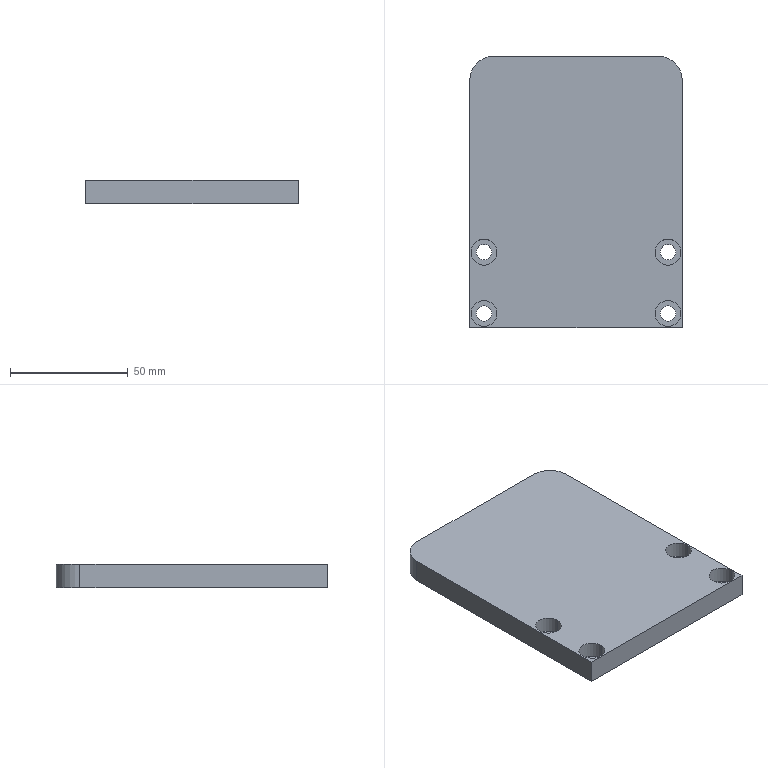Component | SolidWorks | LongSideClampingAssemblyBGeneralAssembly-1_PullFramePlate-0510-1 | 1 solid | 28 faces | box 90 x 115 x 10 mm | volume 100048 mm3 | cylinder 18 | plane 10 | commonest cylinder face diameters 11 x8 6.6 x8 20 x2 | material Q235-A
build123d program:
from build123d import *

# Parameters (mm, degrees)
SKETCH1_W                                          = 90
SKETCH1_H                                          = 115
BOSS_EXTRUDE1_DEPTH                                = 10
HOLE_SIZE_ACCORDING_TO_TYPE_OF_HEX_SOC_D           = 6.6
HOLE_SIZE_ACCORDING_TO_TYPE_OF_HEX_SOC_CBORE_D     = 11
HOLE_SIZE_ACCORDING_TO_TYPE_OF_HEX_SOC_CBORE_DEPTH = 6.8
FILLET1_R                                          = 10


with BuildPart() as part:
    # Sketch1 → Boss-Extrude1 (new body)
    with BuildSketch(Plane.XY):
        Rectangle(SKETCH1_W, SKETCH1_H)
    extrude(amount=BOSS_EXTRUDE1_DEPTH)

    # Hole Size _According to_ Type of Hex Soc (through all)
    with Locations(Plane.XY.offset(10)):
        with Locations((-39, 51.5), (39, 51.5), (-39, 25.5), (39, 25.5)):
            CounterBoreHole(HOLE_SIZE_ACCORDING_TO_TYPE_OF_HEX_SOC_D / 2, HOLE_SIZE_ACCORDING_TO_TYPE_OF_HEX_SOC_CBORE_D / 2, HOLE_SIZE_ACCORDING_TO_TYPE_OF_HEX_SOC_CBORE_DEPTH)

    # Fillet1
    fillet1_edges = [part.edges().sort_by_distance(p)[0] for p in [
        (45, -57.5, 5),
        (-45, -57.5, 5),
    ]]
    fillet(fillet1_edges, radius=FILLET1_R)


solid = part.part

# Placed as in the assembly
solid = solid.moved(Location((-3120.658, -125.109, 3585.5), (0, 0, 180)))
STEP:
#1=COLOUR_RGB('',0.7922,0.8196,0.9333);
#2=FILL_AREA_STYLE_COLOUR('',#1);
#3=FILL_AREA_STYLE('',(#2));
#4=SURFACE_STYLE_FILL_AREA(#3);
#5=SURFACE_SIDE_STYLE('',(#4));
#6=SURFACE_STYLE_USAGE(.BOTH.,#5);
#7=PRESENTATION_STYLE_ASSIGNMENT((#6));
#8=CARTESIAN_POINT('',(-121.109,-6.953,141.287));
#9=VERTEX_POINT('',#8);
#10=CARTESIAN_POINT('',(-121.542,-6.953,141.287));
#11=VERTEX_POINT('',#10);
#12=CARTESIAN_POINT('',(-121.325,-6.953,141.287));
#13=DIRECTION('',(-0.,0.,1.));
#14=DIRECTION('',(-1.,0.,0.));
#15=AXIS2_PLACEMENT_3D('',#12,#13,#14);
#16=CIRCLE('',#15,0.2165);
#17=EDGE_CURVE('',#9,#11,#16,.T.);
#18=ORIENTED_EDGE('',*,*,#17,.F.);
#19=CARTESIAN_POINT('',(-121.109,-6.953,141.555));
#20=VERTEX_POINT('',#19);
#21=CARTESIAN_POINT('',(-121.109,-6.953,141.555));
#22=DIRECTION('',(-0.,0.,1.));
#23=VECTOR('',#22,39.37);
#24=LINE('',#21,#23);
#25=EDGE_CURVE('',#9,#20,#24,.T.);
#26=ORIENTED_EDGE('',*,*,#25,.T.);
#27=CARTESIAN_POINT('',(-121.542,-6.953,141.555));
#28=VERTEX_POINT('',#27);
#29=CARTESIAN_POINT('',(-121.325,-6.953,141.555));
#30=DIRECTION('',(-0.,0.,1.));
#31=DIRECTION('',(-1.,0.,0.));
#32=AXIS2_PLACEMENT_3D('',#29,#30,#31);
#33=CIRCLE('',#32,0.2165);
#34=EDGE_CURVE('',#20,#28,#33,.T.);
#35=ORIENTED_EDGE('',*,*,#34,.T.);
#36=CARTESIAN_POINT('',(-121.542,-6.953,141.555));
#37=DIRECTION('',(-0.,0.,1.));
#38=VECTOR('',#37,39.37);
#39=LINE('',#36,#38);
#40=EDGE_CURVE('',#11,#28,#39,.T.);
#41=ORIENTED_EDGE('',*,*,#40,.F.);
#42=EDGE_LOOP('',(#18,#26,#35,#41));
#43=FACE_OUTER_BOUND('',#42,.T.);
#44=CARTESIAN_POINT('',(-121.325,-6.953,141.555));
#45=DIRECTION('',(-0.,0.,1.));
#46=DIRECTION('',(-1.,0.,0.));
#47=AXIS2_PLACEMENT_3D('',#44,#45,#46);
#48=CYLINDRICAL_SURFACE('',#47,0.2165);
#49=ADVANCED_FACE('',(#43),#48,.F.);
#50=CARTESIAN_POINT('',(-121.195,-6.953,141.161));
#51=VERTEX_POINT('',#50);
#52=CARTESIAN_POINT('',(-121.455,-6.953,141.161));
#53=VERTEX_POINT('',#52);
#54=CARTESIAN_POINT('',(-121.325,-6.953,141.161));
#55=DIRECTION('',(-0.,0.,1.));
#56=DIRECTION('',(-1.,0.,0.));
#57=AXIS2_PLACEMENT_3D('',#54,#55,#56);
#58=CIRCLE('',#57,0.1299);
#59=EDGE_CURVE('',#51,#53,#58,.T.);
#60=ORIENTED_EDGE('',*,*,#59,.F.);
#61=CARTESIAN_POINT('',(-121.195,-6.953,141.287));
#62=VERTEX_POINT('',#61);
#63=CARTESIAN_POINT('',(-121.195,-6.953,141.555));
#64=DIRECTION('',(-0.,0.,1.));
#65=VECTOR('',#64,39.37);
#66=LINE('',#63,#65);
#67=EDGE_CURVE('',#51,#62,#66,.T.);
#68=ORIENTED_EDGE('',*,*,#67,.T.);
#69=CARTESIAN_POINT('',(-121.455,-6.953,141.287));
#70=VERTEX_POINT('',#69);
#71=CARTESIAN_POINT('',(-121.325,-6.953,141.287));
#72=DIRECTION('',(-0.,0.,1.));
#73=DIRECTION('',(-1.,0.,0.));
#74=AXIS2_PLACEMENT_3D('',#71,#72,#73);
#75=CIRCLE('',#74,0.1299);
#76=EDGE_CURVE('',#62,#70,#75,.T.);
#77=ORIENTED_EDGE('',*,*,#76,.T.);
#78=CARTESIAN_POINT('',(-121.455,-6.953,141.555));
#79=DIRECTION('',(-0.,0.,1.));
#80=VECTOR('',#79,39.37);
#81=LINE('',#78,#80);
#82=EDGE_CURVE('',#53,#70,#81,.T.);
#83=ORIENTED_EDGE('',*,*,#82,.F.);
#84=EDGE_LOOP('',(#60,#68,#77,#83));
#85=FACE_OUTER_BOUND('',#84,.T.);
#86=CARTESIAN_POINT('',(-121.325,-6.953,141.555));
#87=DIRECTION('',(-0.,0.,1.));
#88=DIRECTION('',(-1.,0.,0.));
#89=AXIS2_PLACEMENT_3D('',#86,#87,#88);
#90=CYLINDRICAL_SURFACE('',#89,0.1299);
#91=ADVANCED_FACE('',(#85),#90,.F.);
#92=CARTESIAN_POINT('',(-124.179,-6.953,141.287));
#93=VERTEX_POINT('',#92);
#94=CARTESIAN_POINT('',(-124.613,-6.953,141.287));
#95=VERTEX_POINT('',#94);
#96=CARTESIAN_POINT('',(-124.396,-6.953,141.287));
#97=DIRECTION('',(-0.,0.,1.));
#98=DIRECTION('',(-1.,0.,0.));
#99=AXIS2_PLACEMENT_3D('',#96,#97,#98);
#100=CIRCLE('',#99,0.2165);
#101=EDGE_CURVE('',#93,#95,#100,.T.);
#102=ORIENTED_EDGE('',*,*,#101,.F.);
#103=CARTESIAN_POINT('',(-124.179,-6.953,141.555));
#104=VERTEX_POINT('',#103);
#105=CARTESIAN_POINT('',(-124.179,-6.953,141.555));
#106=DIRECTION('',(-0.,0.,1.));
#107=VECTOR('',#106,39.37);
#108=LINE('',#105,#107);
#109=EDGE_CURVE('',#93,#104,#108,.T.);
#110=ORIENTED_EDGE('',*,*,#109,.T.);
#111=CARTESIAN_POINT('',(-124.613,-6.953,141.555));
#112=VERTEX_POINT('',#111);
#113=CARTESIAN_POINT('',(-124.396,-6.953,141.555));
#114=DIRECTION('',(-0.,0.,1.));
#115=DIRECTION('',(-1.,0.,0.));
#116=AXIS2_PLACEMENT_3D('',#113,#114,#115);
#117=CIRCLE('',#116,0.2165);
#118=EDGE_CURVE('',#104,#112,#117,.T.);
#119=ORIENTED_EDGE('',*,*,#118,.T.);
#120=CARTESIAN_POINT('',(-124.613,-6.953,141.555));
#121=DIRECTION('',(-0.,0.,1.));
#122=VECTOR('',#121,39.37);
#123=LINE('',#120,#122);
#124=EDGE_CURVE('',#95,#112,#123,.T.);
#125=ORIENTED_EDGE('',*,*,#124,.F.);
#126=EDGE_LOOP('',(#102,#110,#119,#125));
#127=FACE_OUTER_BOUND('',#126,.T.);
#128=CARTESIAN_POINT('',(-124.396,-6.953,141.555));
#129=DIRECTION('',(-0.,0.,1.));
#130=DIRECTION('',(-1.,0.,0.));
#131=AXIS2_PLACEMENT_3D('',#128,#129,#130);
#132=CYLINDRICAL_SURFACE('',#131,0.2165);
#133=ADVANCED_FACE('',(#127),#132,.F.);
#134=CARTESIAN_POINT('',(-124.266,-6.953,141.161));
#135=VERTEX_POINT('',#134);
#136=CARTESIAN_POINT('',(-124.526,-6.953,141.161));
#137=VERTEX_POINT('',#136);
#138=CARTESIAN_POINT('',(-124.396,-6.953,141.161));
#139=DIRECTION('',(-0.,0.,1.));
#140=DIRECTION('',(-1.,0.,0.));
#141=AXIS2_PLACEMENT_3D('',#138,#139,#140);
#142=CIRCLE('',#141,0.1299);
#143=EDGE_CURVE('',#135,#137,#142,.T.);
#144=ORIENTED_EDGE('',*,*,#143,.F.);
#145=CARTESIAN_POINT('',(-124.266,-6.953,141.287));
#146=VERTEX_POINT('',#145);
#147=CARTESIAN_POINT('',(-124.266,-6.953,141.555));
#148=DIRECTION('',(-0.,0.,1.));
#149=VECTOR('',#148,39.37);
#150=LINE('',#147,#149);
#151=EDGE_CURVE('',#135,#146,#150,.T.);
#152=ORIENTED_EDGE('',*,*,#151,.T.);
#153=CARTESIAN_POINT('',(-124.526,-6.953,141.287));
#154=VERTEX_POINT('',#153);
#155=CARTESIAN_POINT('',(-124.396,-6.953,141.287));
#156=DIRECTION('',(-0.,0.,1.));
#157=DIRECTION('',(-1.,0.,0.));
#158=AXIS2_PLACEMENT_3D('',#155,#156,#157);
#159=CIRCLE('',#158,0.1299);
#160=EDGE_CURVE('',#146,#154,#159,.T.);
#161=ORIENTED_EDGE('',*,*,#160,.T.);
#162=CARTESIAN_POINT('',(-124.526,-6.953,141.555));
#163=DIRECTION('',(-0.,0.,1.));
#164=VECTOR('',#163,39.37);
#165=LINE('',#162,#164);
#166=EDGE_CURVE('',#137,#154,#165,.T.);
#167=ORIENTED_EDGE('',*,*,#166,.F.);
#168=EDGE_LOOP('',(#144,#152,#161,#167));
#169=FACE_OUTER_BOUND('',#168,.T.);
#170=CARTESIAN_POINT('',(-124.396,-6.953,141.555));
#171=DIRECTION('',(-0.,0.,1.));
#172=DIRECTION('',(-1.,0.,0.));
#173=AXIS2_PLACEMENT_3D('',#170,#171,#172);
#174=CYLINDRICAL_SURFACE('',#173,0.1299);
#175=ADVANCED_FACE('',(#169),#174,.F.);
#176=CARTESIAN_POINT('',(-121.109,-5.929,141.287));
#177=VERTEX_POINT('',#176);
#178=CARTESIAN_POINT('',(-121.542,-5.929,141.287));
#179=VERTEX_POINT('',#178);
#180=CARTESIAN_POINT('',(-121.325,-5.929,141.287));
#181=DIRECTION('',(-0.,0.,1.));
#182=DIRECTION('',(-1.,0.,0.));
#183=AXIS2_PLACEMENT_3D('',#180,#181,#182);
#184=CIRCLE('',#183,0.2165);
#185=EDGE_CURVE('',#177,#179,#184,.T.);
#186=ORIENTED_EDGE('',*,*,#185,.F.);
#187=CARTESIAN_POINT('',(-121.109,-5.929,141.555));
#188=VERTEX_POINT('',#187);
#189=CARTESIAN_POINT('',(-121.109,-5.929,141.555));
#190=DIRECTION('',(-0.,0.,1.));
#191=VECTOR('',#190,39.37);
#192=LINE('',#189,#191);
#193=EDGE_CURVE('',#177,#188,#192,.T.);
#194=ORIENTED_EDGE('',*,*,#193,.T.);
#195=CARTESIAN_POINT('',(-121.542,-5.929,141.555));
#196=VERTEX_POINT('',#195);
#197=CARTESIAN_POINT('',(-121.325,-5.929,141.555));
#198=DIRECTION('',(-0.,0.,1.));
#199=DIRECTION('',(-1.,0.,0.));
#200=AXIS2_PLACEMENT_3D('',#197,#198,#199);
#201=CIRCLE('',#200,0.2165);
#202=EDGE_CURVE('',#188,#196,#201,.T.);
#203=ORIENTED_EDGE('',*,*,#202,.T.);
#204=CARTESIAN_POINT('',(-121.542,-5.929,141.555));
#205=DIRECTION('',(-0.,0.,1.));
#206=VECTOR('',#205,39.37);
#207=LINE('',#204,#206);
#208=EDGE_CURVE('',#179,#196,#207,.T.);
#209=ORIENTED_EDGE('',*,*,#208,.F.);
#210=EDGE_LOOP('',(#186,#194,#203,#209));
#211=FACE_OUTER_BOUND('',#210,.T.);
#212=CARTESIAN_POINT('',(-121.325,-5.929,141.555));
#213=DIRECTION('',(-0.,0.,1.));
#214=DIRECTION('',(-1.,0.,0.));
#215=AXIS2_PLACEMENT_3D('',#212,#213,#214);
#216=CYLINDRICAL_SURFACE('',#215,0.2165);
#217=ADVANCED_FACE('',(#211),#216,.F.);
#218=CARTESIAN_POINT('',(-121.195,-5.929,141.161));
#219=VERTEX_POINT('',#218);
#220=CARTESIAN_POINT('',(-121.455,-5.929,141.161));
#221=VERTEX_POINT('',#220);
#222=CARTESIAN_POINT('',(-121.325,-5.929,141.161));
#223=DIRECTION('',(-0.,0.,1.));
#224=DIRECTION('',(-1.,0.,0.));
#225=AXIS2_PLACEMENT_3D('',#222,#223,#224);
#226=CIRCLE('',#225,0.1299);
#227=EDGE_CURVE('',#219,#221,#226,.T.);
#228=ORIENTED_EDGE('',*,*,#227,.F.);
#229=CARTESIAN_POINT('',(-121.195,-5.929,141.287));
#230=VERTEX_POINT('',#229);
#231=CARTESIAN_POINT('',(-121.195,-5.929,141.555));
#232=DIRECTION('',(-0.,0.,1.));
#233=VECTOR('',#232,39.37);
#234=LINE('',#231,#233);
#235=EDGE_CURVE('',#219,#230,#234,.T.);
#236=ORIENTED_EDGE('',*,*,#235,.T.);
#237=CARTESIAN_POINT('',(-121.455,-5.929,141.287));
#238=VERTEX_POINT('',#237);
#239=CARTESIAN_POINT('',(-121.325,-5.929,141.287));
#240=DIRECTION('',(-0.,0.,1.));
#241=DIRECTION('',(-1.,0.,0.));
#242=AXIS2_PLACEMENT_3D('',#239,#240,#241);
#243=CIRCLE('',#242,0.1299);
#244=EDGE_CURVE('',#230,#238,#243,.T.);
#245=ORIENTED_EDGE('',*,*,#244,.T.);
#246=CARTESIAN_POINT('',(-121.455,-5.929,141.555));
#247=DIRECTION('',(-0.,0.,1.));
#248=VECTOR('',#247,39.37);
#249=LINE('',#246,#248);
#250=EDGE_CURVE('',#221,#238,#249,.T.);
#251=ORIENTED_EDGE('',*,*,#250,.F.);
#252=EDGE_LOOP('',(#228,#236,#245,#251));
#253=FACE_OUTER_BOUND('',#252,.T.);
#254=CARTESIAN_POINT('',(-121.325,-5.929,141.555));
#255=DIRECTION('',(-0.,0.,1.));
#256=DIRECTION('',(-1.,0.,0.));
#257=AXIS2_PLACEMENT_3D('',#254,#255,#256);
#258=CYLINDRICAL_SURFACE('',#257,0.1299);
#259=ADVANCED_FACE('',(#253),#258,.F.);
#260=CARTESIAN_POINT('',(-124.179,-5.929,141.287));
#261=VERTEX_POINT('',#260);
#262=CARTESIAN_POINT('',(-124.613,-5.929,141.287));
#263=VERTEX_POINT('',#262);
#264=CARTESIAN_POINT('',(-124.396,-5.929,141.287));
#265=DIRECTION('',(-0.,0.,1.));
#266=DIRECTION('',(-1.,0.,0.));
#267=AXIS2_PLACEMENT_3D('',#264,#265,#266);
#268=CIRCLE('',#267,0.2165);
#269=EDGE_CURVE('',#261,#263,#268,.T.);
#270=ORIENTED_EDGE('',*,*,#269,.F.);
#271=CARTESIAN_POINT('',(-124.179,-5.929,141.555));
#272=VERTEX_POINT('',#271);
#273=CARTESIAN_POINT('',(-124.179,-5.929,141.555));
#274=DIRECTION('',(-0.,0.,1.));
#275=VECTOR('',#274,39.37);
#276=LINE('',#273,#275);
#277=EDGE_CURVE('',#261,#272,#276,.T.);
#278=ORIENTED_EDGE('',*,*,#277,.T.);
#279=CARTESIAN_POINT('',(-124.613,-5.929,141.555));
#280=VERTEX_POINT('',#279);
#281=CARTESIAN_POINT('',(-124.396,-5.929,141.555));
#282=DIRECTION('',(-0.,0.,1.));
#283=DIRECTION('',(-1.,0.,0.));
#284=AXIS2_PLACEMENT_3D('',#281,#282,#283);
#285=CIRCLE('',#284,0.2165);
#286=EDGE_CURVE('',#272,#280,#285,.T.);
#287=ORIENTED_EDGE('',*,*,#286,.T.);
#288=CARTESIAN_POINT('',(-124.613,-5.929,141.555));
#289=DIRECTION('',(-0.,0.,1.));
#290=VECTOR('',#289,39.37);
#291=LINE('',#288,#290);
#292=EDGE_CURVE('',#263,#280,#291,.T.);
#293=ORIENTED_EDGE('',*,*,#292,.F.);
#294=EDGE_LOOP('',(#270,#278,#287,#293));
#295=FACE_OUTER_BOUND('',#294,.T.);
#296=CARTESIAN_POINT('',(-124.396,-5.929,141.555));
#297=DIRECTION('',(-0.,0.,1.));
#298=DIRECTION('',(-1.,0.,0.));
#299=AXIS2_PLACEMENT_3D('',#296,#297,#298);
#300=CYLINDRICAL_SURFACE('',#299,0.2165);
#301=ADVANCED_FACE('',(#295),#300,.F.);
#302=CARTESIAN_POINT('',(-124.266,-5.929,141.161));
#303=VERTEX_POINT('',#302);
#304=CARTESIAN_POINT('',(-124.526,-5.929,141.161));
#305=VERTEX_POINT('',#304);
#306=CARTESIAN_POINT('',(-124.396,-5.929,141.161));
#307=DIRECTION('',(-0.,0.,1.));
#308=DIRECTION('',(-1.,0.,0.));
#309=AXIS2_PLACEMENT_3D('',#306,#307,#308);
#310=CIRCLE('',#309,0.1299);
#311=EDGE_CURVE('',#303,#305,#310,.T.);
#312=ORIENTED_EDGE('',*,*,#311,.F.);
#313=CARTESIAN_POINT('',(-124.266,-5.929,141.287));
#314=VERTEX_POINT('',#313);
#315=CARTESIAN_POINT('',(-124.266,-5.929,141.555));
#316=DIRECTION('',(-0.,0.,1.));
#317=VECTOR('',#316,39.37);
#318=LINE('',#315,#317);
#319=EDGE_CURVE('',#303,#314,#318,.T.);
#320=ORIENTED_EDGE('',*,*,#319,.T.);
#321=CARTESIAN_POINT('',(-124.526,-5.929,141.287));
#322=VERTEX_POINT('',#321);
#323=CARTESIAN_POINT('',(-124.396,-5.929,141.287));
#324=DIRECTION('',(-0.,0.,1.));
#325=DIRECTION('',(-1.,0.,0.));
#326=AXIS2_PLACEMENT_3D('',#323,#324,#325);
#327=CIRCLE('',#326,0.1299);
#328=EDGE_CURVE('',#314,#322,#327,.T.);
#329=ORIENTED_EDGE('',*,*,#328,.T.);
#330=CARTESIAN_POINT('',(-124.526,-5.929,141.555));
#331=DIRECTION('',(-0.,0.,1.));
#332=VECTOR('',#331,39.37);
#333=LINE('',#330,#332);
#334=EDGE_CURVE('',#305,#322,#333,.T.);
#335=ORIENTED_EDGE('',*,*,#334,.F.);
#336=EDGE_LOOP('',(#312,#320,#329,#335));
#337=FACE_OUTER_BOUND('',#336,.T.);
#338=CARTESIAN_POINT('',(-124.396,-5.929,141.555));
#339=DIRECTION('',(-0.,0.,1.));
#340=DIRECTION('',(-1.,0.,0.));
#341=AXIS2_PLACEMENT_3D('',#338,#339,#340);
#342=CYLINDRICAL_SURFACE('',#341,0.1299);
#343=ADVANCED_FACE('',(#337),#342,.F.);
#344=CARTESIAN_POINT('',(-124.632,-3.055,141.555));
#345=VERTEX_POINT('',#344);
#346=CARTESIAN_POINT('',(-124.632,-7.189,141.555));
#347=VERTEX_POINT('',#346);
#348=CARTESIAN_POINT('',(-124.632,-2.662,141.555));
#349=DIRECTION('',(-0.,-1.,0.));
#350=VECTOR('',#349,39.37);
#351=LINE('',#348,#350);
#352=EDGE_CURVE('',#345,#347,#351,.T.);
#353=ORIENTED_EDGE('',*,*,#352,.F.);
#354=CARTESIAN_POINT('',(-124.632,-3.055,141.161));
#355=VERTEX_POINT('',#354);
#356=CARTESIAN_POINT('',(-124.632,-3.055,141.555));
#357=DIRECTION('',(0.,-0.,-1.));
#358=VECTOR('',#357,39.37);
#359=LINE('',#356,#358);
#360=EDGE_CURVE('',#345,#355,#359,.T.);
#361=ORIENTED_EDGE('',*,*,#360,.T.);
#362=CARTESIAN_POINT('',(-124.632,-7.189,141.161));
#363=VERTEX_POINT('',#362);
#364=CARTESIAN_POINT('',(-124.632,-2.662,141.161));
#365=DIRECTION('',(-0.,-1.,0.));
#366=VECTOR('',#365,39.37);
#367=LINE('',#364,#366);
#368=EDGE_CURVE('',#355,#363,#367,.T.);
#369=ORIENTED_EDGE('',*,*,#368,.T.);
#370=CARTESIAN_POINT('',(-124.632,-7.189,141.555));
#371=DIRECTION('',(0.,-0.,-1.));
#372=VECTOR('',#371,39.37);
#373=LINE('',#370,#372);
#374=EDGE_CURVE('',#347,#363,#373,.T.);
#375=ORIENTED_EDGE('',*,*,#374,.F.);
#376=EDGE_LOOP('',(#353,#361,#369,#375));
#377=FACE_OUTER_BOUND('',#376,.T.);
#378=CARTESIAN_POINT('',(-124.632,-2.662,141.555));
#379=DIRECTION('',(1.,-0.,0.));
#380=DIRECTION('',(-0.,0.,1.));
#381=AXIS2_PLACEMENT_3D('',#378,#379,#380);
#382=PLANE('',#381);
#383=ADVANCED_FACE('',(#377),#382,.F.);
#384=CARTESIAN_POINT('',(-121.089,-7.189,141.161));
#385=VERTEX_POINT('',#384);
#386=CARTESIAN_POINT('',(-121.089,-7.189,141.161));
#387=DIRECTION('',(1.,-0.,0.));
#388=VECTOR('',#387,39.37);
#389=LINE('',#386,#388);
#390=EDGE_CURVE('',#363,#385,#389,.T.);
#391=ORIENTED_EDGE('',*,*,#390,.T.);
#392=CARTESIAN_POINT('',(-121.089,-7.189,141.555));
#393=VERTEX_POINT('',#392);
#394=CARTESIAN_POINT('',(-121.089,-7.189,141.555));
#395=DIRECTION('',(0.,-0.,-1.));
#396=VECTOR('',#395,39.37);
#397=LINE('',#394,#396);
#398=EDGE_CURVE('',#393,#385,#397,.T.);
#399=ORIENTED_EDGE('',*,*,#398,.F.);
#400=CARTESIAN_POINT('',(-121.089,-7.189,141.555));
#401=DIRECTION('',(1.,-0.,0.));
#402=VECTOR('',#401,39.37);
#403=LINE('',#400,#402);
#404=EDGE_CURVE('',#347,#393,#403,.T.);
#405=ORIENTED_EDGE('',*,*,#404,.F.);
#406=ORIENTED_EDGE('',*,*,#374,.T.);
#407=EDGE_LOOP('',(#391,#399,#405,#406));
#408=FACE_OUTER_BOUND('',#407,.T.);
#409=CARTESIAN_POINT('',(-121.089,-7.189,141.555));
#410=DIRECTION('',(0.,1.,-0.));
#411=DIRECTION('',(0.,-0.,-1.));
#412=AXIS2_PLACEMENT_3D('',#409,#410,#411);
#413=PLANE('',#412);
#414=ADVANCED_FACE('',(#408),#413,.F.);
#415=CARTESIAN_POINT('',(-121.089,-3.055,141.161));
#416=VERTEX_POINT('',#415);
#417=CARTESIAN_POINT('',(-121.089,-2.662,141.161));
#418=DIRECTION('',(0.,1.,-0.));
#419=VECTOR('',#418,39.37);
#420=LINE('',#417,#419);
#421=EDGE_CURVE('',#385,#416,#420,.T.);
#422=ORIENTED_EDGE('',*,*,#421,.T.);
#423=CARTESIAN_POINT('',(-121.089,-3.055,141.555));
#424=VERTEX_POINT('',#423);
#425=CARTESIAN_POINT('',(-121.089,-3.055,141.555));
#426=DIRECTION('',(-0.,0.,1.));
#427=VECTOR('',#426,39.37);
#428=LINE('',#425,#427);
#429=EDGE_CURVE('',#416,#424,#428,.T.);
#430=ORIENTED_EDGE('',*,*,#429,.T.);
#431=CARTESIAN_POINT('',(-121.089,-2.662,141.555));
#432=DIRECTION('',(0.,1.,-0.));
#433=VECTOR('',#432,39.37);
#434=LINE('',#431,#433);
#435=EDGE_CURVE('',#393,#424,#434,.T.);
#436=ORIENTED_EDGE('',*,*,#435,.F.);
#437=ORIENTED_EDGE('',*,*,#398,.T.);
#438=EDGE_LOOP('',(#422,#430,#436,#437));
#439=FACE_OUTER_BOUND('',#438,.T.);
#440=CARTESIAN_POINT('',(-121.089,-2.662,141.555));
#441=DIRECTION('',(-1.,0.,-0.));
#442=DIRECTION('',(0.,-0.,-1.));
#443=AXIS2_PLACEMENT_3D('',#440,#441,#442);
#444=PLANE('',#443);
#445=ADVANCED_FACE('',(#439),#444,.F.);
#446=CARTESIAN_POINT('',(-121.483,-2.662,141.555));
#447=VERTEX_POINT('',#446);
#448=CARTESIAN_POINT('',(-124.239,-2.662,141.555));
#449=VERTEX_POINT('',#448);
#450=CARTESIAN_POINT('',(-121.089,-2.662,141.555));
#451=DIRECTION('',(-1.,0.,-0.));
#452=VECTOR('',#451,39.37);
#453=LINE('',#450,#452);
#454=EDGE_CURVE('',#447,#449,#453,.T.);
#455=ORIENTED_EDGE('',*,*,#454,.F.);
#456=CARTESIAN_POINT('',(-121.483,-2.662,141.161));
#457=VERTEX_POINT('',#456);
#458=CARTESIAN_POINT('',(-121.483,-2.662,141.555));
#459=DIRECTION('',(0.,-0.,-1.));
#460=VECTOR('',#459,39.37);
#461=LINE('',#458,#460);
#462=EDGE_CURVE('',#447,#457,#461,.T.);
#463=ORIENTED_EDGE('',*,*,#462,.T.);
#464=CARTESIAN_POINT('',(-124.239,-2.662,141.161));
#465=VERTEX_POINT('',#464);
#466=CARTESIAN_POINT('',(-121.089,-2.662,141.161));
#467=DIRECTION('',(-1.,0.,-0.));
#468=VECTOR('',#467,39.37);
#469=LINE('',#466,#468);
#470=EDGE_CURVE('',#457,#465,#469,.T.);
#471=ORIENTED_EDGE('',*,*,#470,.T.);
#472=CARTESIAN_POINT('',(-124.239,-2.662,141.555));
#473=DIRECTION('',(-0.,0.,1.));
#474=VECTOR('',#473,39.37);
#475=LINE('',#472,#474);
#476=EDGE_CURVE('',#465,#449,#475,.T.);
#477=ORIENTED_EDGE('',*,*,#476,.T.);
#478=EDGE_LOOP('',(#455,#463,#471,#477));
#479=FACE_OUTER_BOUND('',#478,.T.);
#480=CARTESIAN_POINT('',(-121.089,-2.662,141.555));
#481=DIRECTION('',(-0.,-1.,0.));
#482=DIRECTION('',(-0.,0.,1.));
#483=AXIS2_PLACEMENT_3D('',#480,#481,#482);
#484=PLANE('',#483);
#485=ADVANCED_FACE('',(#479),#484,.F.);
#486=CARTESIAN_POINT('',(-121.325,-6.953,141.555));
#487=DIRECTION('',(-0.,0.,1.));
#488=DIRECTION('',(-1.,0.,0.));
#489=AXIS2_PLACEMENT_3D('',#486,#487,#488);
#490=CIRCLE('',#489,0.2165);
#491=EDGE_CURVE('',#28,#20,#490,.T.);
#492=ORIENTED_EDGE('',*,*,#491,.F.);
#493=ORIENTED_EDGE('',*,*,#34,.F.);
#494=EDGE_LOOP('',(#492,#493));
#495=FACE_BOUND('',#494,.T.);
#496=CARTESIAN_POINT('',(-124.396,-6.953,141.555));
#497=DIRECTION('',(-0.,0.,1.));
#498=DIRECTION('',(-1.,0.,0.));
#499=AXIS2_PLACEMENT_3D('',#496,#497,#498);
#500=CIRCLE('',#499,0.2165);
#501=EDGE_CURVE('',#112,#104,#500,.T.);
#502=ORIENTED_EDGE('',*,*,#501,.F.);
#503=ORIENTED_EDGE('',*,*,#118,.F.);
#504=EDGE_LOOP('',(#502,#503));
#505=FACE_BOUND('',#504,.T.);
#506=CARTESIAN_POINT('',(-121.325,-5.929,141.555));
#507=DIRECTION('',(-0.,0.,1.));
#508=DIRECTION('',(-1.,0.,0.));
#509=AXIS2_PLACEMENT_3D('',#506,#507,#508);
#510=CIRCLE('',#509,0.2165);
#511=EDGE_CURVE('',#196,#188,#510,.T.);
#512=ORIENTED_EDGE('',*,*,#511,.F.);
#513=ORIENTED_EDGE('',*,*,#202,.F.);
#514=EDGE_LOOP('',(#512,#513));
#515=FACE_BOUND('',#514,.T.);
#516=CARTESIAN_POINT('',(-124.396,-5.929,141.555));
#517=DIRECTION('',(-0.,0.,1.));
#518=DIRECTION('',(-1.,0.,0.));
#519=AXIS2_PLACEMENT_3D('',#516,#517,#518);
#520=CIRCLE('',#519,0.2165);
#521=EDGE_CURVE('',#280,#272,#520,.T.);
#522=ORIENTED_EDGE('',*,*,#521,.F.);
#523=ORIENTED_EDGE('',*,*,#286,.F.);
#524=EDGE_LOOP('',(#522,#523));
#525=FACE_BOUND('',#524,.T.);
#526=ORIENTED_EDGE('',*,*,#435,.T.);
#527=CARTESIAN_POINT('',(-121.483,-3.055,141.555));
#528=DIRECTION('',(-0.,0.,1.));
#529=DIRECTION('',(1.,-0.,0.));
#530=AXIS2_PLACEMENT_3D('',#527,#528,#529);
#531=CIRCLE('',#530,0.3937);
#532=EDGE_CURVE('',#424,#447,#531,.T.);
#533=ORIENTED_EDGE('',*,*,#532,.T.);
#534=ORIENTED_EDGE('',*,*,#454,.T.);
#535=CARTESIAN_POINT('',(-124.239,-3.055,141.555));
#536=DIRECTION('',(-0.,0.,1.));
#537=DIRECTION('',(1.,-0.,0.));
#538=AXIS2_PLACEMENT_3D('',#535,#536,#537);
#539=CIRCLE('',#538,0.3937);
#540=EDGE_CURVE('',#449,#345,#539,.T.);
#541=ORIENTED_EDGE('',*,*,#540,.T.);
#542=ORIENTED_EDGE('',*,*,#352,.T.);
#543=ORIENTED_EDGE('',*,*,#404,.T.);
#544=EDGE_LOOP('',(#526,#533,#534,#541,#542,#543));
#545=FACE_OUTER_BOUND('',#544,.T.);
#546=CARTESIAN_POINT('',(-122.861,-4.926,141.555));
#547=DIRECTION('',(0.,-0.,-1.));
#548=DIRECTION('',(1.,-0.,0.));
#549=AXIS2_PLACEMENT_3D('',#546,#547,#548);
#550=PLANE('',#549);
#551=ADVANCED_FACE('',(#495,#505,#515,#525,#545),#550,.F.);
#552=CARTESIAN_POINT('',(-121.325,-6.953,141.161));
#553=DIRECTION('',(-0.,0.,1.));
#554=DIRECTION('',(-1.,0.,0.));
#555=AXIS2_PLACEMENT_3D('',#552,#553,#554);
#556=CIRCLE('',#555,0.1299);
#557=EDGE_CURVE('',#53,#51,#556,.T.);
#558=ORIENTED_EDGE('',*,*,#557,.T.);
#559=ORIENTED_EDGE('',*,*,#59,.T.);
#560=EDGE_LOOP('',(#558,#559));
#561=FACE_BOUND('',#560,.T.);
#562=CARTESIAN_POINT('',(-124.396,-6.953,141.161));
#563=DIRECTION('',(-0.,0.,1.));
#564=DIRECTION('',(-1.,0.,0.));
#565=AXIS2_PLACEMENT_3D('',#562,#563,#564);
#566=CIRCLE('',#565,0.1299);
#567=EDGE_CURVE('',#137,#135,#566,.T.);
#568=ORIENTED_EDGE('',*,*,#567,.T.);
#569=ORIENTED_EDGE('',*,*,#143,.T.);
#570=EDGE_LOOP('',(#568,#569));
#571=FACE_BOUND('',#570,.T.);
#572=CARTESIAN_POINT('',(-121.325,-5.929,141.161));
#573=DIRECTION('',(-0.,0.,1.));
#574=DIRECTION('',(-1.,0.,0.));
#575=AXIS2_PLACEMENT_3D('',#572,#573,#574);
#576=CIRCLE('',#575,0.1299);
#577=EDGE_CURVE('',#221,#219,#576,.T.);
#578=ORIENTED_EDGE('',*,*,#577,.T.);
#579=ORIENTED_EDGE('',*,*,#227,.T.);
#580=EDGE_LOOP('',(#578,#579));
#581=FACE_BOUND('',#580,.T.);
#582=CARTESIAN_POINT('',(-124.396,-5.929,141.161));
#583=DIRECTION('',(-0.,0.,1.));
#584=DIRECTION('',(-1.,0.,0.));
#585=AXIS2_PLACEMENT_3D('',#582,#583,#584);
#586=CIRCLE('',#585,0.1299);
#587=EDGE_CURVE('',#305,#303,#586,.T.);
#588=ORIENTED_EDGE('',*,*,#587,.T.);
#589=ORIENTED_EDGE('',*,*,#311,.T.);
#590=EDGE_LOOP('',(#588,#589));
#591=FACE_BOUND('',#590,.T.);
#592=ORIENTED_EDGE('',*,*,#470,.F.);
#593=CARTESIAN_POINT('',(-121.483,-3.055,141.161));
#594=DIRECTION('',(0.,-0.,-1.));
#595=DIRECTION('',(1.,-0.,0.));
#596=AXIS2_PLACEMENT_3D('',#593,#594,#595);
#597=CIRCLE('',#596,0.3937);
#598=EDGE_CURVE('',#457,#416,#597,.T.);
#599=ORIENTED_EDGE('',*,*,#598,.T.);
#600=ORIENTED_EDGE('',*,*,#421,.F.);
#601=ORIENTED_EDGE('',*,*,#390,.F.);
#602=ORIENTED_EDGE('',*,*,#368,.F.);
#603=CARTESIAN_POINT('',(-124.239,-3.055,141.161));
#604=DIRECTION('',(0.,-0.,-1.));
#605=DIRECTION('',(1.,-0.,0.));
#606=AXIS2_PLACEMENT_3D('',#603,#604,#605);
#607=CIRCLE('',#606,0.3937);
#608=EDGE_CURVE('',#355,#465,#607,.T.);
#609=ORIENTED_EDGE('',*,*,#608,.T.);
#610=EDGE_LOOP('',(#592,#599,#600,#601,#602,#609));
#611=FACE_OUTER_BOUND('',#610,.T.);
#612=CARTESIAN_POINT('',(-122.861,-4.926,141.161));
#613=DIRECTION('',(0.,-0.,-1.));
#614=DIRECTION('',(1.,-0.,0.));
#615=AXIS2_PLACEMENT_3D('',#612,#613,#614);
#616=PLANE('',#615);
#617=ADVANCED_FACE('',(#561,#571,#581,#591,#611),#616,.T.);
#618=ORIENTED_EDGE('',*,*,#319,.F.);
#619=ORIENTED_EDGE('',*,*,#587,.F.);
#620=ORIENTED_EDGE('',*,*,#334,.T.);
#621=CARTESIAN_POINT('',(-124.396,-5.929,141.287));
#622=DIRECTION('',(-0.,0.,1.));
#623=DIRECTION('',(-1.,0.,0.));
#624=AXIS2_PLACEMENT_3D('',#621,#622,#623);
#625=CIRCLE('',#624,0.1299);
#626=EDGE_CURVE('',#322,#314,#625,.T.);
#627=ORIENTED_EDGE('',*,*,#626,.T.);
#628=EDGE_LOOP('',(#618,#619,#620,#627));
#629=FACE_OUTER_BOUND('',#628,.T.);
#630=CARTESIAN_POINT('',(-124.396,-5.929,141.555));
#631=DIRECTION('',(-0.,0.,1.));
#632=DIRECTION('',(-1.,0.,0.));
#633=AXIS2_PLACEMENT_3D('',#630,#631,#632);
#634=CYLINDRICAL_SURFACE('',#633,0.1299);
#635=ADVANCED_FACE('',(#629),#634,.F.);
#636=ORIENTED_EDGE('',*,*,#626,.F.);
#637=ORIENTED_EDGE('',*,*,#328,.F.);
#638=EDGE_LOOP('',(#636,#637));
#639=FACE_BOUND('',#638,.T.);
#640=CARTESIAN_POINT('',(-124.396,-5.929,141.287));
#641=DIRECTION('',(-0.,0.,1.));
#642=DIRECTION('',(-1.,0.,0.));
#643=AXIS2_PLACEMENT_3D('',#640,#641,#642);
#644=CIRCLE('',#643,0.2165);
#645=EDGE_CURVE('',#263,#261,#644,.T.);
#646=ORIENTED_EDGE('',*,*,#645,.T.);
#647=ORIENTED_EDGE('',*,*,#269,.T.);
#648=EDGE_LOOP('',(#646,#647));
#649=FACE_OUTER_BOUND('',#648,.T.);
#650=CARTESIAN_POINT('',(-124.526,-5.929,141.287));
#651=DIRECTION('',(0.,-0.,-1.));
#652=DIRECTION('',(1.,-0.,0.));
#653=AXIS2_PLACEMENT_3D('',#650,#651,#652);
#654=PLANE('',#653);
#655=ADVANCED_FACE('',(#639,#649),#654,.F.);
#656=ORIENTED_EDGE('',*,*,#277,.F.);
#657=ORIENTED_EDGE('',*,*,#645,.F.);
#658=ORIENTED_EDGE('',*,*,#292,.T.);
#659=ORIENTED_EDGE('',*,*,#521,.T.);
#660=EDGE_LOOP('',(#656,#657,#658,#659));
#661=FACE_OUTER_BOUND('',#660,.T.);
#662=CARTESIAN_POINT('',(-124.396,-5.929,141.555));
#663=DIRECTION('',(-0.,0.,1.));
#664=DIRECTION('',(-1.,0.,0.));
#665=AXIS2_PLACEMENT_3D('',#662,#663,#664);
#666=CYLINDRICAL_SURFACE('',#665,0.2165);
#667=ADVANCED_FACE('',(#661),#666,.F.);
#668=ORIENTED_EDGE('',*,*,#235,.F.);
#669=ORIENTED_EDGE('',*,*,#577,.F.);
#670=ORIENTED_EDGE('',*,*,#250,.T.);
#671=CARTESIAN_POINT('',(-121.325,-5.929,141.287));
#672=DIRECTION('',(-0.,0.,1.));
#673=DIRECTION('',(-1.,0.,0.));
#674=AXIS2_PLACEMENT_3D('',#671,#672,#673);
#675=CIRCLE('',#674,0.1299);
#676=EDGE_CURVE('',#238,#230,#675,.T.);
#677=ORIENTED_EDGE('',*,*,#676,.T.);
#678=EDGE_LOOP('',(#668,#669,#670,#677));
#679=FACE_OUTER_BOUND('',#678,.T.);
#680=CARTESIAN_POINT('',(-121.325,-5.929,141.555));
#681=DIRECTION('',(-0.,0.,1.));
#682=DIRECTION('',(-1.,0.,0.));
#683=AXIS2_PLACEMENT_3D('',#680,#681,#682);
#684=CYLINDRICAL_SURFACE('',#683,0.1299);
#685=ADVANCED_FACE('',(#679),#684,.F.);
#686=ORIENTED_EDGE('',*,*,#676,.F.);
#687=ORIENTED_EDGE('',*,*,#244,.F.);
#688=EDGE_LOOP('',(#686,#687));
#689=FACE_BOUND('',#688,.T.);
#690=CARTESIAN_POINT('',(-121.325,-5.929,141.287));
#691=DIRECTION('',(-0.,0.,1.));
#692=DIRECTION('',(-1.,0.,0.));
#693=AXIS2_PLACEMENT_3D('',#690,#691,#692);
#694=CIRCLE('',#693,0.2165);
#695=EDGE_CURVE('',#179,#177,#694,.T.);
#696=ORIENTED_EDGE('',*,*,#695,.T.);
#697=ORIENTED_EDGE('',*,*,#185,.T.);
#698=EDGE_LOOP('',(#696,#697));
#699=FACE_OUTER_BOUND('',#698,.T.);
#700=CARTESIAN_POINT('',(-121.455,-5.929,141.287));
#701=DIRECTION('',(0.,-0.,-1.));
#702=DIRECTION('',(1.,-0.,0.));
#703=AXIS2_PLACEMENT_3D('',#700,#701,#702);
#704=PLANE('',#703);
#705=ADVANCED_FACE('',(#689,#699),#704,.F.);
#706=ORIENTED_EDGE('',*,*,#193,.F.);
#707=ORIENTED_EDGE('',*,*,#695,.F.);
#708=ORIENTED_EDGE('',*,*,#208,.T.);
#709=ORIENTED_EDGE('',*,*,#511,.T.);
#710=EDGE_LOOP('',(#706,#707,#708,#709));
#711=FACE_OUTER_BOUND('',#710,.T.);
#712=CARTESIAN_POINT('',(-121.325,-5.929,141.555));
#713=DIRECTION('',(-0.,0.,1.));
#714=DIRECTION('',(-1.,0.,0.));
#715=AXIS2_PLACEMENT_3D('',#712,#713,#714);
#716=CYLINDRICAL_SURFACE('',#715,0.2165);
#717=ADVANCED_FACE('',(#711),#716,.F.);
#718=ORIENTED_EDGE('',*,*,#151,.F.);
#719=ORIENTED_EDGE('',*,*,#567,.F.);
#720=ORIENTED_EDGE('',*,*,#166,.T.);
#721=CARTESIAN_POINT('',(-124.396,-6.953,141.287));
#722=DIRECTION('',(-0.,0.,1.));
#723=DIRECTION('',(-1.,0.,0.));
#724=AXIS2_PLACEMENT_3D('',#721,#722,#723);
#725=CIRCLE('',#724,0.1299);
#726=EDGE_CURVE('',#154,#146,#725,.T.);
#727=ORIENTED_EDGE('',*,*,#726,.T.);
#728=EDGE_LOOP('',(#718,#719,#720,#727));
#729=FACE_OUTER_BOUND('',#728,.T.);
#730=CARTESIAN_POINT('',(-124.396,-6.953,141.555));
#731=DIRECTION('',(-0.,0.,1.));
#732=DIRECTION('',(-1.,0.,0.));
#733=AXIS2_PLACEMENT_3D('',#730,#731,#732);
#734=CYLINDRICAL_SURFACE('',#733,0.1299);
#735=ADVANCED_FACE('',(#729),#734,.F.);
#736=ORIENTED_EDGE('',*,*,#726,.F.);
#737=ORIENTED_EDGE('',*,*,#160,.F.);
#738=EDGE_LOOP('',(#736,#737));
#739=FACE_BOUND('',#738,.T.);
#740=CARTESIAN_POINT('',(-124.396,-6.953,141.287));
#741=DIRECTION('',(-0.,0.,1.));
#742=DIRECTION('',(-1.,0.,0.));
#743=AXIS2_PLACEMENT_3D('',#740,#741,#742);
#744=CIRCLE('',#743,0.2165);
#745=EDGE_CURVE('',#95,#93,#744,.T.);
#746=ORIENTED_EDGE('',*,*,#745,.T.);
#747=ORIENTED_EDGE('',*,*,#101,.T.);
#748=EDGE_LOOP('',(#746,#747));
#749=FACE_OUTER_BOUND('',#748,.T.);
#750=CARTESIAN_POINT('',(-124.526,-6.953,141.287));
#751=DIRECTION('',(0.,-0.,-1.));
#752=DIRECTION('',(1.,-0.,0.));
#753=AXIS2_PLACEMENT_3D('',#750,#751,#752);
#754=PLANE('',#753);
#755=ADVANCED_FACE('',(#739,#749),#754,.F.);
#756=ORIENTED_EDGE('',*,*,#109,.F.);
#757=ORIENTED_EDGE('',*,*,#745,.F.);
#758=ORIENTED_EDGE('',*,*,#124,.T.);
#759=ORIENTED_EDGE('',*,*,#501,.T.);
#760=EDGE_LOOP('',(#756,#757,#758,#759));
#761=FACE_OUTER_BOUND('',#760,.T.);
#762=CARTESIAN_POINT('',(-124.396,-6.953,141.555));
#763=DIRECTION('',(-0.,0.,1.));
#764=DIRECTION('',(-1.,0.,0.));
#765=AXIS2_PLACEMENT_3D('',#762,#763,#764);
#766=CYLINDRICAL_SURFACE('',#765,0.2165);
#767=ADVANCED_FACE('',(#761),#766,.F.);
#768=ORIENTED_EDGE('',*,*,#67,.F.);
#769=ORIENTED_EDGE('',*,*,#557,.F.);
#770=ORIENTED_EDGE('',*,*,#82,.T.);
#771=CARTESIAN_POINT('',(-121.325,-6.953,141.287));
#772=DIRECTION('',(-0.,0.,1.));
#773=DIRECTION('',(-1.,0.,0.));
#774=AXIS2_PLACEMENT_3D('',#771,#772,#773);
#775=CIRCLE('',#774,0.1299);
#776=EDGE_CURVE('',#70,#62,#775,.T.);
#777=ORIENTED_EDGE('',*,*,#776,.T.);
#778=EDGE_LOOP('',(#768,#769,#770,#777));
#779=FACE_OUTER_BOUND('',#778,.T.);
#780=CARTESIAN_POINT('',(-121.325,-6.953,141.555));
#781=DIRECTION('',(-0.,0.,1.));
#782=DIRECTION('',(-1.,0.,0.));
#783=AXIS2_PLACEMENT_3D('',#780,#781,#782);
#784=CYLINDRICAL_SURFACE('',#783,0.1299);
#785=ADVANCED_FACE('',(#779),#784,.F.);
#786=ORIENTED_EDGE('',*,*,#776,.F.);
#787=ORIENTED_EDGE('',*,*,#76,.F.);
#788=EDGE_LOOP('',(#786,#787));
#789=FACE_BOUND('',#788,.T.);
#790=CARTESIAN_POINT('',(-121.325,-6.953,141.287));
#791=DIRECTION('',(-0.,0.,1.));
#792=DIRECTION('',(-1.,0.,0.));
#793=AXIS2_PLACEMENT_3D('',#790,#791,#792);
#794=CIRCLE('',#793,0.2165);
#795=EDGE_CURVE('',#11,#9,#794,.T.);
#796=ORIENTED_EDGE('',*,*,#795,.T.);
#797=ORIENTED_EDGE('',*,*,#17,.T.);
#798=EDGE_LOOP('',(#796,#797));
#799=FACE_OUTER_BOUND('',#798,.T.);
#800=CARTESIAN_POINT('',(-121.455,-6.953,141.287));
#801=DIRECTION('',(0.,-0.,-1.));
#802=DIRECTION('',(1.,-0.,0.));
#803=AXIS2_PLACEMENT_3D('',#800,#801,#802);
#804=PLANE('',#803);
#805=ADVANCED_FACE('',(#789,#799),#804,.F.);
#806=ORIENTED_EDGE('',*,*,#25,.F.);
#807=ORIENTED_EDGE('',*,*,#795,.F.);
#808=ORIENTED_EDGE('',*,*,#40,.T.);
#809=ORIENTED_EDGE('',*,*,#491,.T.);
#810=EDGE_LOOP('',(#806,#807,#808,#809));
#811=FACE_OUTER_BOUND('',#810,.T.);
#812=CARTESIAN_POINT('',(-121.325,-6.953,141.555));
#813=DIRECTION('',(-0.,0.,1.));
#814=DIRECTION('',(-1.,0.,0.));
#815=AXIS2_PLACEMENT_3D('',#812,#813,#814);
#816=CYLINDRICAL_SURFACE('',#815,0.2165);
#817=ADVANCED_FACE('',(#811),#816,.F.);
#818=ORIENTED_EDGE('',*,*,#532,.F.);
#819=ORIENTED_EDGE('',*,*,#429,.F.);
#820=ORIENTED_EDGE('',*,*,#598,.F.);
#821=ORIENTED_EDGE('',*,*,#462,.F.);
#822=EDGE_LOOP('',(#818,#819,#820,#821));
#823=FACE_OUTER_BOUND('',#822,.T.);
#824=CARTESIAN_POINT('',(-121.483,-3.055,141.555));
#825=DIRECTION('',(0.,-0.,-1.));
#826=DIRECTION('',(1.,-0.,0.));
#827=AXIS2_PLACEMENT_3D('',#824,#825,#826);
#828=CYLINDRICAL_SURFACE('',#827,0.3937);
#829=ADVANCED_FACE('',(#823),#828,.T.);
#830=ORIENTED_EDGE('',*,*,#540,.F.);
#831=ORIENTED_EDGE('',*,*,#476,.F.);
#832=ORIENTED_EDGE('',*,*,#608,.F.);
#833=ORIENTED_EDGE('',*,*,#360,.F.);
#834=EDGE_LOOP('',(#830,#831,#832,#833));
#835=FACE_OUTER_BOUND('',#834,.T.);
#836=CARTESIAN_POINT('',(-124.239,-3.055,141.555));
#837=DIRECTION('',(0.,-0.,-1.));
#838=DIRECTION('',(1.,-0.,0.));
#839=AXIS2_PLACEMENT_3D('',#836,#837,#838);
#840=CYLINDRICAL_SURFACE('',#839,0.3937);
#841=ADVANCED_FACE('',(#835),#840,.T.);
#842=CLOSED_SHELL('',(#49,#91,#133,#175,#217,#259,#301,#343,#383,#414,#445,#485,#551,#617,#635,#655,#667,#685,#705,#717,#735,#755,#767,#785,#805,#817,#829,#841));
#843=MANIFOLD_SOLID_BREP('',#842);
#844=STYLED_ITEM('',(#7),#843);
#845=(LENGTH_UNIT()NAMED_UNIT(*)SI_UNIT($,.METRE.));
#846=LENGTH_MEASURE_WITH_UNIT(LENGTH_MEASURE(0.0254),#845);
#847=DIMENSIONAL_EXPONENTS(1.,0.,0.,0.,0.,0.,0.);
#848=(CONVERSION_BASED_UNIT('',#846)LENGTH_UNIT()NAMED_UNIT(#847));
#849=UNCERTAINTY_MEASURE_WITH_UNIT(LENGTH_MEASURE(0.00001),#848,'','');
#850=(NAMED_UNIT(*)PLANE_ANGLE_UNIT()SI_UNIT($,.RADIAN.));
#851=(NAMED_UNIT(*)SI_UNIT($,.STERADIAN.)SOLID_ANGLE_UNIT());
#852=(GEOMETRIC_REPRESENTATION_CONTEXT(3)GLOBAL_UNCERTAINTY_ASSIGNED_CONTEXT((#849))GLOBAL_UNIT_ASSIGNED_CONTEXT((#848,#850,#851))REPRESENTATION_CONTEXT('',''));
#853=MECHANICAL_DESIGN_GEOMETRIC_PRESENTATION_REPRESENTATION('',(#844),#852);
#854=CARTESIAN_POINT('',(0.,0.,0.));
#855=DIRECTION('',(0.,0.,1.));
#856=DIRECTION('',(1.,0.,0.));
#857=AXIS2_PLACEMENT_3D('',#854,#855,#856);
#858=(LENGTH_UNIT()NAMED_UNIT(*)SI_UNIT($,.METRE.));
#859=LENGTH_MEASURE_WITH_UNIT(LENGTH_MEASURE(0.0254),#858);
#860=DIMENSIONAL_EXPONENTS(1.,0.,0.,0.,0.,0.,0.);
#861=(CONVERSION_BASED_UNIT('',#859)LENGTH_UNIT()NAMED_UNIT(#860));
#862=UNCERTAINTY_MEASURE_WITH_UNIT(LENGTH_MEASURE(0.00001),#861,'','');
#863=(NAMED_UNIT(*)PLANE_ANGLE_UNIT()SI_UNIT($,.RADIAN.));
#864=(NAMED_UNIT(*)SI_UNIT($,.STERADIAN.)SOLID_ANGLE_UNIT());
#865=(GEOMETRIC_REPRESENTATION_CONTEXT(3)GLOBAL_UNCERTAINTY_ASSIGNED_CONTEXT((#862))GLOBAL_UNIT_ASSIGNED_CONTEXT((#861,#863,#864))REPRESENTATION_CONTEXT('',''));
#866=ADVANCED_BREP_SHAPE_REPRESENTATION('',(#843,#857),#865);
#867=PRESENTATION_LAYER_ASSIGNMENT('','',(#844));